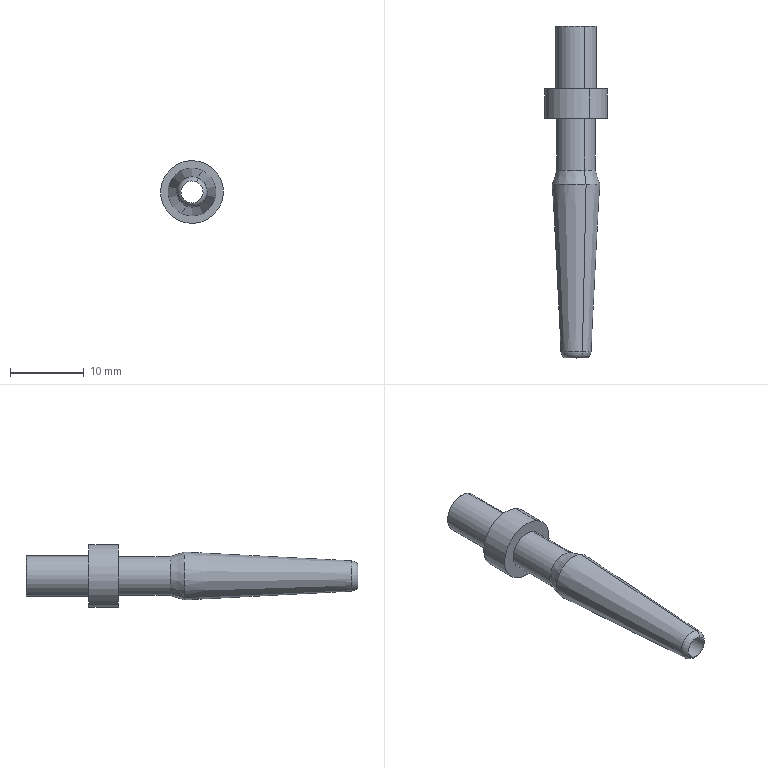Component | SolidWorks | WireFeedingNozzle-1 | 1 solid | 19 faces | box 8.5 x 44.89 x 8.5 mm | volume 831 mm3 | cylinder 8 | cone 6 | plane 3 | torus 2 | commonest cylinder face diameters 3 x2 5.5 x2 8.5 x2 5.274 x2
build123d program:
from build123d import *

# Parameters (mm, degrees)
FILLET3_R          = 1
CUT_EXTRUDE1_REACH = 47.4
SKETCH2_R          = 1.5
CHAMFER1_SIZE      = 0.08


with BuildPart() as part:
    # Sketch1 → Revolve1 (revolve)
    with BuildSketch(Plane.XY, mode=Mode.PRIVATE) as revolve1_sk:
        Polygon((-15.381, 0), (29.619, 0), (29.619, 2), (6.04, 3.236), (4.119, 2.637), (-2.881, 2.637), (-2.881, 4.25), (-6.881, 4.25), (-6.881, 2.75), (-15.381, 2.75), align=None)
    revolve(revolve1_sk.sketch.rotate(Axis((-15.381, 0, 0), (1, 0, 0)), 90), axis=Axis((-15.381, 0, 0), (1, 0, 0)))

    # Fillet3
    fillet3_edges = [part.edges().sort_by_distance(p)[0] for p in [
        (29.619, 0, -2),
    ]]
    fillet(fillet3_edges, radius=FILLET3_R)

    # Sketch2 → Cut-Extrude1 (cut, up to next)
    with BuildSketch(Plane.ZY.offset(15.381), mode=Mode.PRIVATE) as cut_extrude1_sk1:
        Circle(SKETCH2_R)
    cut_extrude1_tool1 = extrude(cut_extrude1_sk1.sketch, amount=-CUT_EXTRUDE1_REACH, mode=Mode.PRIVATE) & part.part
    add(cut_extrude1_tool1.solids().sort_by_distance((-15.381, 0, 0))[0], mode=Mode.SUBTRACT)

    # Chamfer1
    chamfer1_edges = [part.edges().sort_by_distance(p)[0] for p in [
        (-15.381, 0, -2.75),
    ]]
    chamfer(chamfer1_edges, length=CHAMFER1_SIZE)


solid = part.part

# Placed as in the assembly
solid = solid.moved(Location((-5.981, -114.875, 160), (0, 0, -90)))
STEP:
#1=CARTESIAN_POINT('',(-0.1912,-3.917,6.395));
#2=VERTEX_POINT('',#1);
#3=CARTESIAN_POINT('',(-0.2797,-3.917,6.204));
#4=VERTEX_POINT('',#3);
#5=CARTESIAN_POINT('',(-0.2355,-3.917,6.299));
#6=DIRECTION('',(0.,1.,0.));
#7=DIRECTION('',(-0.421,0.,-0.9071));
#8=AXIS2_PLACEMENT_3D('',#5,#6,#7);
#9=CIRCLE('',#8,0.1051);
#10=EDGE_CURVE('',#2,#4,#9,.T.);
#11=ORIENTED_EDGE('',*,*,#10,.F.);
#12=CARTESIAN_POINT('',(-0.1899,-3.92,6.397));
#13=VERTEX_POINT('',#12);
#14=CARTESIAN_POINT('',(-0.1912,-3.917,6.395));
#15=DIRECTION('',(0.2977,-0.7071,0.6414));
#16=VECTOR('',#15,39.37);
#17=LINE('',#14,#16);
#18=EDGE_CURVE('',#2,#13,#17,.T.);
#19=ORIENTED_EDGE('',*,*,#18,.T.);
#20=CARTESIAN_POINT('',(-0.281,-3.92,6.201));
#21=VERTEX_POINT('',#20);
#22=CARTESIAN_POINT('',(-0.2355,-3.92,6.299));
#23=DIRECTION('',(-0.,-1.,-0.));
#24=DIRECTION('',(-0.421,0.,-0.9071));
#25=AXIS2_PLACEMENT_3D('',#22,#23,#24);
#26=CIRCLE('',#25,0.1083);
#27=EDGE_CURVE('',#21,#13,#26,.T.);
#28=ORIENTED_EDGE('',*,*,#27,.F.);
#29=CARTESIAN_POINT('',(-0.2797,-3.917,6.204));
#30=DIRECTION('',(-0.2977,-0.7071,-0.6414));
#31=VECTOR('',#30,39.37);
#32=LINE('',#29,#31);
#33=EDGE_CURVE('',#4,#21,#32,.T.);
#34=ORIENTED_EDGE('',*,*,#33,.F.);
#35=EDGE_LOOP('',(#11,#19,#28,#34));
#36=FACE_OUTER_BOUND('',#35,.T.);
#37=CARTESIAN_POINT('',(-0.2355,-3.917,6.299));
#38=DIRECTION('',(-0.,-1.,-0.));
#39=DIRECTION('',(-0.421,0.,-0.9071));
#40=AXIS2_PLACEMENT_3D('',#37,#38,#39);
#41=CONICAL_SURFACE('',#40,0.1051,0.7854);
#42=ADVANCED_FACE('',(#36),#41,.T.);
#43=CARTESIAN_POINT('',(-0.2603,-5.685,6.246));
#44=VERTEX_POINT('',#43);
#45=CARTESIAN_POINT('',(-0.2106,-5.685,6.353));
#46=VERTEX_POINT('',#45);
#47=CARTESIAN_POINT('',(-0.2355,-5.685,6.299));
#48=DIRECTION('',(0.,1.,0.));
#49=DIRECTION('',(0.421,0.,0.9071));
#50=AXIS2_PLACEMENT_3D('',#47,#48,#49);
#51=CIRCLE('',#50,0.05906);
#52=EDGE_CURVE('',#44,#46,#51,.T.);
#53=ORIENTED_EDGE('',*,*,#52,.F.);
#54=CARTESIAN_POINT('',(-0.2603,-3.917,6.246));
#55=VERTEX_POINT('',#54);
#56=CARTESIAN_POINT('',(-0.2603,-5.689,6.246));
#57=DIRECTION('',(0.,1.,0.));
#58=VECTOR('',#57,39.37);
#59=LINE('',#56,#58);
#60=EDGE_CURVE('',#44,#55,#59,.T.);
#61=ORIENTED_EDGE('',*,*,#60,.T.);
#62=CARTESIAN_POINT('',(-0.2106,-3.917,6.353));
#63=VERTEX_POINT('',#62);
#64=CARTESIAN_POINT('',(-0.2355,-3.917,6.299));
#65=DIRECTION('',(0.,1.,0.));
#66=DIRECTION('',(0.421,0.,0.9071));
#67=AXIS2_PLACEMENT_3D('',#64,#65,#66);
#68=CIRCLE('',#67,0.05906);
#69=EDGE_CURVE('',#55,#63,#68,.T.);
#70=ORIENTED_EDGE('',*,*,#69,.T.);
#71=CARTESIAN_POINT('',(-0.2106,-5.689,6.353));
#72=DIRECTION('',(0.,1.,0.));
#73=VECTOR('',#72,39.37);
#74=LINE('',#71,#73);
#75=EDGE_CURVE('',#46,#63,#74,.T.);
#76=ORIENTED_EDGE('',*,*,#75,.F.);
#77=EDGE_LOOP('',(#53,#61,#70,#76));
#78=FACE_OUTER_BOUND('',#77,.T.);
#79=CARTESIAN_POINT('',(-0.2355,-5.689,6.299));
#80=DIRECTION('',(0.,1.,0.));
#81=DIRECTION('',(0.421,0.,0.9071));
#82=AXIS2_PLACEMENT_3D('',#79,#80,#81);
#83=CYLINDRICAL_SURFACE('',#82,0.05906);
#84=ADVANCED_FACE('',(#78),#83,.F.);
#85=CARTESIAN_POINT('',(-0.2355,-5.685,6.299));
#86=DIRECTION('',(0.,1.,0.));
#87=DIRECTION('',(0.421,0.,0.9071));
#88=AXIS2_PLACEMENT_3D('',#85,#86,#87);
#89=CIRCLE('',#88,0.05906);
#90=EDGE_CURVE('',#46,#44,#89,.T.);
#91=ORIENTED_EDGE('',*,*,#90,.T.);
#92=CARTESIAN_POINT('',(-0.2694,-5.651,6.226));
#93=VERTEX_POINT('',#92);
#94=CARTESIAN_POINT('',(-0.2529,-5.649,6.262));
#95=DIRECTION('',(0.9071,-0.,-0.421));
#96=DIRECTION('',(-0.421,0.,-0.9071));
#97=AXIS2_PLACEMENT_3D('',#94,#95,#96);
#98=CIRCLE('',#97,0.03937);
#99=EDGE_CURVE('',#44,#93,#98,.T.);
#100=ORIENTED_EDGE('',*,*,#99,.T.);
#101=CARTESIAN_POINT('',(-0.2015,-5.651,6.372));
#102=VERTEX_POINT('',#101);
#103=CARTESIAN_POINT('',(-0.2355,-5.651,6.299));
#104=DIRECTION('',(0.,1.,0.));
#105=DIRECTION('',(-0.421,0.,-0.9071));
#106=AXIS2_PLACEMENT_3D('',#103,#104,#105);
#107=CIRCLE('',#106,0.0807);
#108=EDGE_CURVE('',#102,#93,#107,.T.);
#109=ORIENTED_EDGE('',*,*,#108,.F.);
#110=CARTESIAN_POINT('',(-0.218,-5.649,6.337));
#111=DIRECTION('',(-0.9071,0.,0.421));
#112=DIRECTION('',(0.421,0.,0.9071));
#113=AXIS2_PLACEMENT_3D('',#110,#111,#112);
#114=CIRCLE('',#113,0.03937);
#115=EDGE_CURVE('',#46,#102,#114,.T.);
#116=ORIENTED_EDGE('',*,*,#115,.F.);
#117=EDGE_LOOP('',(#91,#100,#109,#116));
#118=FACE_OUTER_BOUND('',#117,.T.);
#119=CARTESIAN_POINT('',(-0.2355,-5.649,6.299));
#120=DIRECTION('',(0.,1.,0.));
#121=DIRECTION('',(0.421,-0.,0.9071));
#122=AXIS2_PLACEMENT_3D('',#119,#120,#121);
#123=TOROIDAL_SURFACE('',#122,0.04138,0.03937);
#124=ADVANCED_FACE('',(#118),#123,.T.);
#125=CARTESIAN_POINT('',(-0.1899,-4.252,6.397));
#126=VERTEX_POINT('',#125);
#127=CARTESIAN_POINT('',(-0.281,-4.252,6.201));
#128=VERTEX_POINT('',#127);
#129=CARTESIAN_POINT('',(-0.2355,-4.252,6.299));
#130=DIRECTION('',(0.,1.,0.));
#131=DIRECTION('',(0.421,0.,0.9071));
#132=AXIS2_PLACEMENT_3D('',#129,#130,#131);
#133=CIRCLE('',#132,0.1083);
#134=EDGE_CURVE('',#126,#128,#133,.T.);
#135=ORIENTED_EDGE('',*,*,#134,.T.);
#136=CARTESIAN_POINT('',(-0.281,-3.917,6.201));
#137=DIRECTION('',(0.,1.,0.));
#138=VECTOR('',#137,39.37);
#139=LINE('',#136,#138);
#140=EDGE_CURVE('',#128,#21,#139,.T.);
#141=ORIENTED_EDGE('',*,*,#140,.T.);
#142=ORIENTED_EDGE('',*,*,#27,.T.);
#143=CARTESIAN_POINT('',(-0.1899,-3.917,6.397));
#144=DIRECTION('',(0.,1.,0.));
#145=VECTOR('',#144,39.37);
#146=LINE('',#143,#145);
#147=EDGE_CURVE('',#126,#13,#146,.T.);
#148=ORIENTED_EDGE('',*,*,#147,.F.);
#149=EDGE_LOOP('',(#135,#141,#142,#148));
#150=FACE_OUTER_BOUND('',#149,.T.);
#151=CARTESIAN_POINT('',(-0.2355,-3.917,6.299));
#152=DIRECTION('',(0.,1.,0.));
#153=DIRECTION('',(0.421,0.,0.9071));
#154=AXIS2_PLACEMENT_3D('',#151,#152,#153);
#155=CYLINDRICAL_SURFACE('',#154,0.1083);
#156=ADVANCED_FACE('',(#150),#155,.T.);
#157=CARTESIAN_POINT('',(-0.165,-4.409,6.451));
#158=VERTEX_POINT('',#157);
#159=CARTESIAN_POINT('',(-0.3059,-4.409,6.147));
#160=VERTEX_POINT('',#159);
#161=CARTESIAN_POINT('',(-0.2355,-4.409,6.299));
#162=DIRECTION('',(0.,1.,0.));
#163=DIRECTION('',(0.421,0.,0.9071));
#164=AXIS2_PLACEMENT_3D('',#161,#162,#163);
#165=CIRCLE('',#164,0.1673);
#166=EDGE_CURVE('',#158,#160,#165,.T.);
#167=ORIENTED_EDGE('',*,*,#166,.T.);
#168=CARTESIAN_POINT('',(-0.3059,-4.252,6.147));
#169=VERTEX_POINT('',#168);
#170=CARTESIAN_POINT('',(-0.3059,-3.917,6.147));
#171=DIRECTION('',(0.,1.,0.));
#172=VECTOR('',#171,39.37);
#173=LINE('',#170,#172);
#174=EDGE_CURVE('',#160,#169,#173,.T.);
#175=ORIENTED_EDGE('',*,*,#174,.T.);
#176=CARTESIAN_POINT('',(-0.165,-4.252,6.451));
#177=VERTEX_POINT('',#176);
#178=CARTESIAN_POINT('',(-0.2355,-4.252,6.299));
#179=DIRECTION('',(0.,1.,0.));
#180=DIRECTION('',(0.421,0.,0.9071));
#181=AXIS2_PLACEMENT_3D('',#178,#179,#180);
#182=CIRCLE('',#181,0.1673);
#183=EDGE_CURVE('',#177,#169,#182,.T.);
#184=ORIENTED_EDGE('',*,*,#183,.F.);
#185=CARTESIAN_POINT('',(-0.165,-3.917,6.451));
#186=DIRECTION('',(0.,1.,0.));
#187=VECTOR('',#186,39.37);
#188=LINE('',#185,#187);
#189=EDGE_CURVE('',#158,#177,#188,.T.);
#190=ORIENTED_EDGE('',*,*,#189,.F.);
#191=EDGE_LOOP('',(#167,#175,#184,#190));
#192=FACE_OUTER_BOUND('',#191,.T.);
#193=CARTESIAN_POINT('',(-0.2355,-3.917,6.299));
#194=DIRECTION('',(0.,1.,0.));
#195=DIRECTION('',(0.421,0.,0.9071));
#196=AXIS2_PLACEMENT_3D('',#193,#194,#195);
#197=CYLINDRICAL_SURFACE('',#196,0.1673);
#198=ADVANCED_FACE('',(#192),#197,.T.);
#199=CARTESIAN_POINT('',(-0.1918,-4.685,6.393));
#200=VERTEX_POINT('',#199);
#201=CARTESIAN_POINT('',(-0.2792,-4.685,6.205));
#202=VERTEX_POINT('',#201);
#203=CARTESIAN_POINT('',(-0.2355,-4.685,6.299));
#204=DIRECTION('',(0.,1.,0.));
#205=DIRECTION('',(0.421,0.,0.9071));
#206=AXIS2_PLACEMENT_3D('',#203,#204,#205);
#207=CIRCLE('',#206,0.1038);
#208=EDGE_CURVE('',#200,#202,#207,.T.);
#209=ORIENTED_EDGE('',*,*,#208,.T.);
#210=CARTESIAN_POINT('',(-0.2792,-4.409,6.205));
#211=VERTEX_POINT('',#210);
#212=CARTESIAN_POINT('',(-0.2792,-3.917,6.205));
#213=DIRECTION('',(0.,1.,0.));
#214=VECTOR('',#213,39.37);
#215=LINE('',#212,#214);
#216=EDGE_CURVE('',#202,#211,#215,.T.);
#217=ORIENTED_EDGE('',*,*,#216,.T.);
#218=CARTESIAN_POINT('',(-0.1918,-4.409,6.393));
#219=VERTEX_POINT('',#218);
#220=CARTESIAN_POINT('',(-0.2355,-4.409,6.299));
#221=DIRECTION('',(0.,1.,0.));
#222=DIRECTION('',(0.421,0.,0.9071));
#223=AXIS2_PLACEMENT_3D('',#220,#221,#222);
#224=CIRCLE('',#223,0.1038);
#225=EDGE_CURVE('',#219,#211,#224,.T.);
#226=ORIENTED_EDGE('',*,*,#225,.F.);
#227=CARTESIAN_POINT('',(-0.1918,-3.917,6.393));
#228=DIRECTION('',(0.,1.,0.));
#229=VECTOR('',#228,39.37);
#230=LINE('',#227,#229);
#231=EDGE_CURVE('',#200,#219,#230,.T.);
#232=ORIENTED_EDGE('',*,*,#231,.F.);
#233=EDGE_LOOP('',(#209,#217,#226,#232));
#234=FACE_OUTER_BOUND('',#233,.T.);
#235=CARTESIAN_POINT('',(-0.2355,-3.917,6.299));
#236=DIRECTION('',(0.,1.,0.));
#237=DIRECTION('',(0.421,0.,0.9071));
#238=AXIS2_PLACEMENT_3D('',#235,#236,#237);
#239=CYLINDRICAL_SURFACE('',#238,0.1038);
#240=ADVANCED_FACE('',(#234),#239,.T.);
#241=ORIENTED_EDGE('',*,*,#208,.F.);
#242=CARTESIAN_POINT('',(-0.1818,-4.76,6.415));
#243=VERTEX_POINT('',#242);
#244=CARTESIAN_POINT('',(-0.1818,-4.76,6.415));
#245=DIRECTION('',(0.1253,-0.9547,0.27));
#246=VECTOR('',#245,39.37);
#247=LINE('',#244,#246);
#248=EDGE_CURVE('',#200,#243,#247,.T.);
#249=ORIENTED_EDGE('',*,*,#248,.T.);
#250=CARTESIAN_POINT('',(-0.2891,-4.76,6.184));
#251=VERTEX_POINT('',#250);
#252=CARTESIAN_POINT('',(-0.2355,-4.76,6.299));
#253=DIRECTION('',(0.,1.,0.));
#254=DIRECTION('',(0.421,0.,0.9071));
#255=AXIS2_PLACEMENT_3D('',#252,#253,#254);
#256=CIRCLE('',#255,0.1274);
#257=EDGE_CURVE('',#243,#251,#256,.T.);
#258=ORIENTED_EDGE('',*,*,#257,.T.);
#259=CARTESIAN_POINT('',(-0.2891,-4.76,6.184));
#260=DIRECTION('',(-0.1253,-0.9547,-0.27));
#261=VECTOR('',#260,39.37);
#262=LINE('',#259,#261);
#263=EDGE_CURVE('',#202,#251,#262,.T.);
#264=ORIENTED_EDGE('',*,*,#263,.F.);
#265=EDGE_LOOP('',(#241,#249,#258,#264));
#266=FACE_OUTER_BOUND('',#265,.T.);
#267=CARTESIAN_POINT('',(-0.2355,-4.76,6.299));
#268=DIRECTION('',(-0.,-1.,-0.));
#269=DIRECTION('',(-0.421,0.,-0.9071));
#270=AXIS2_PLACEMENT_3D('',#267,#268,#269);
#271=CONICAL_SURFACE('',#270,0.1274,0.3023);
#272=ADVANCED_FACE('',(#266),#271,.T.);
#273=ORIENTED_EDGE('',*,*,#108,.T.);
#274=CARTESIAN_POINT('',(-0.2686,-5.689,6.228));
#275=DIRECTION('',(-0.02203,0.9986,-0.04747));
#276=VECTOR('',#275,39.37);
#277=LINE('',#274,#276);
#278=EDGE_CURVE('',#93,#251,#277,.T.);
#279=ORIENTED_EDGE('',*,*,#278,.T.);
#280=ORIENTED_EDGE('',*,*,#257,.F.);
#281=CARTESIAN_POINT('',(-0.2023,-5.689,6.371));
#282=DIRECTION('',(0.02203,0.9986,0.04747));
#283=VECTOR('',#282,39.37);
#284=LINE('',#281,#283);
#285=EDGE_CURVE('',#102,#243,#284,.T.);
#286=ORIENTED_EDGE('',*,*,#285,.F.);
#287=EDGE_LOOP('',(#273,#279,#280,#286));
#288=FACE_OUTER_BOUND('',#287,.T.);
#289=CARTESIAN_POINT('',(-0.2355,-5.689,6.299));
#290=DIRECTION('',(0.,1.,0.));
#291=DIRECTION('',(0.421,0.,0.9071));
#292=AXIS2_PLACEMENT_3D('',#289,#290,#291);
#293=CONICAL_SURFACE('',#292,0.07874,0.05236);
#294=ADVANCED_FACE('',(#288),#293,.T.);
#295=CARTESIAN_POINT('',(-0.2355,-3.917,6.299));
#296=DIRECTION('',(0.,1.,0.));
#297=DIRECTION('',(-0.421,0.,-0.9071));
#298=AXIS2_PLACEMENT_3D('',#295,#296,#297);
#299=CIRCLE('',#298,0.1051);
#300=EDGE_CURVE('',#4,#2,#299,.T.);
#301=ORIENTED_EDGE('',*,*,#300,.T.);
#302=ORIENTED_EDGE('',*,*,#10,.T.);
#303=EDGE_LOOP('',(#301,#302));
#304=FACE_OUTER_BOUND('',#303,.T.);
#305=CARTESIAN_POINT('',(-0.2355,-3.917,6.299));
#306=DIRECTION('',(0.,1.,0.));
#307=DIRECTION('',(0.421,0.,0.9071));
#308=AXIS2_PLACEMENT_3D('',#305,#306,#307);
#309=CIRCLE('',#308,0.05906);
#310=EDGE_CURVE('',#63,#55,#309,.T.);
#311=ORIENTED_EDGE('',*,*,#310,.F.);
#312=ORIENTED_EDGE('',*,*,#69,.F.);
#313=EDGE_LOOP('',(#311,#312));
#314=FACE_BOUND('',#313,.T.);
#315=CARTESIAN_POINT('',(-0.1373,-3.917,6.254));
#316=DIRECTION('',(-0.,-1.,-0.));
#317=DIRECTION('',(-0.421,0.,-0.9071));
#318=AXIS2_PLACEMENT_3D('',#315,#316,#317);
#319=PLANE('',#318);
#320=ADVANCED_FACE('',(#304,#314),#319,.F.);
#321=ORIENTED_EDGE('',*,*,#278,.F.);
#322=CARTESIAN_POINT('',(-0.2355,-5.651,6.299));
#323=DIRECTION('',(0.,1.,0.));
#324=DIRECTION('',(-0.421,0.,-0.9071));
#325=AXIS2_PLACEMENT_3D('',#322,#323,#324);
#326=CIRCLE('',#325,0.0807);
#327=EDGE_CURVE('',#93,#102,#326,.T.);
#328=ORIENTED_EDGE('',*,*,#327,.T.);
#329=ORIENTED_EDGE('',*,*,#285,.T.);
#330=CARTESIAN_POINT('',(-0.2355,-4.76,6.299));
#331=DIRECTION('',(0.,1.,0.));
#332=DIRECTION('',(0.421,0.,0.9071));
#333=AXIS2_PLACEMENT_3D('',#330,#331,#332);
#334=CIRCLE('',#333,0.1274);
#335=EDGE_CURVE('',#251,#243,#334,.T.);
#336=ORIENTED_EDGE('',*,*,#335,.F.);
#337=EDGE_LOOP('',(#321,#328,#329,#336));
#338=FACE_OUTER_BOUND('',#337,.T.);
#339=CARTESIAN_POINT('',(-0.2355,-5.689,6.299));
#340=DIRECTION('',(0.,1.,0.));
#341=DIRECTION('',(0.421,0.,0.9071));
#342=AXIS2_PLACEMENT_3D('',#339,#340,#341);
#343=CONICAL_SURFACE('',#342,0.07874,0.05236);
#344=ADVANCED_FACE('',(#338),#343,.T.);
#345=ORIENTED_EDGE('',*,*,#248,.F.);
#346=CARTESIAN_POINT('',(-0.2355,-4.685,6.299));
#347=DIRECTION('',(0.,1.,0.));
#348=DIRECTION('',(0.421,0.,0.9071));
#349=AXIS2_PLACEMENT_3D('',#346,#347,#348);
#350=CIRCLE('',#349,0.1038);
#351=EDGE_CURVE('',#202,#200,#350,.T.);
#352=ORIENTED_EDGE('',*,*,#351,.F.);
#353=ORIENTED_EDGE('',*,*,#263,.T.);
#354=ORIENTED_EDGE('',*,*,#335,.T.);
#355=EDGE_LOOP('',(#345,#352,#353,#354));
#356=FACE_OUTER_BOUND('',#355,.T.);
#357=CARTESIAN_POINT('',(-0.2355,-4.76,6.299));
#358=DIRECTION('',(-0.,-1.,-0.));
#359=DIRECTION('',(-0.421,0.,-0.9071));
#360=AXIS2_PLACEMENT_3D('',#357,#358,#359);
#361=CONICAL_SURFACE('',#360,0.1274,0.3023);
#362=ADVANCED_FACE('',(#356),#361,.T.);
#363=ORIENTED_EDGE('',*,*,#216,.F.);
#364=ORIENTED_EDGE('',*,*,#351,.T.);
#365=ORIENTED_EDGE('',*,*,#231,.T.);
#366=CARTESIAN_POINT('',(-0.2355,-4.409,6.299));
#367=DIRECTION('',(0.,1.,0.));
#368=DIRECTION('',(0.421,0.,0.9071));
#369=AXIS2_PLACEMENT_3D('',#366,#367,#368);
#370=CIRCLE('',#369,0.1038);
#371=EDGE_CURVE('',#211,#219,#370,.T.);
#372=ORIENTED_EDGE('',*,*,#371,.F.);
#373=EDGE_LOOP('',(#363,#364,#365,#372));
#374=FACE_OUTER_BOUND('',#373,.T.);
#375=CARTESIAN_POINT('',(-0.2355,-3.917,6.299));
#376=DIRECTION('',(0.,1.,0.));
#377=DIRECTION('',(0.421,0.,0.9071));
#378=AXIS2_PLACEMENT_3D('',#375,#376,#377);
#379=CYLINDRICAL_SURFACE('',#378,0.1038);
#380=ADVANCED_FACE('',(#374),#379,.T.);
#381=ORIENTED_EDGE('',*,*,#166,.F.);
#382=CARTESIAN_POINT('',(-0.2355,-4.409,6.299));
#383=DIRECTION('',(0.,1.,0.));
#384=DIRECTION('',(0.421,0.,0.9071));
#385=AXIS2_PLACEMENT_3D('',#382,#383,#384);
#386=CIRCLE('',#385,0.1673);
#387=EDGE_CURVE('',#160,#158,#386,.T.);
#388=ORIENTED_EDGE('',*,*,#387,.F.);
#389=EDGE_LOOP('',(#381,#388));
#390=FACE_OUTER_BOUND('',#389,.T.);
#391=ORIENTED_EDGE('',*,*,#225,.T.);
#392=ORIENTED_EDGE('',*,*,#371,.T.);
#393=EDGE_LOOP('',(#391,#392));
#394=FACE_BOUND('',#393,.T.);
#395=CARTESIAN_POINT('',(-0.1413,-4.409,6.256));
#396=DIRECTION('',(0.,1.,0.));
#397=DIRECTION('',(0.421,-0.,0.9071));
#398=AXIS2_PLACEMENT_3D('',#395,#396,#397);
#399=PLANE('',#398);
#400=ADVANCED_FACE('',(#390,#394),#399,.F.);
#401=ORIENTED_EDGE('',*,*,#174,.F.);
#402=ORIENTED_EDGE('',*,*,#387,.T.);
#403=ORIENTED_EDGE('',*,*,#189,.T.);
#404=CARTESIAN_POINT('',(-0.2355,-4.252,6.299));
#405=DIRECTION('',(0.,1.,0.));
#406=DIRECTION('',(0.421,0.,0.9071));
#407=AXIS2_PLACEMENT_3D('',#404,#405,#406);
#408=CIRCLE('',#407,0.1673);
#409=EDGE_CURVE('',#169,#177,#408,.T.);
#410=ORIENTED_EDGE('',*,*,#409,.F.);
#411=EDGE_LOOP('',(#401,#402,#403,#410));
#412=FACE_OUTER_BOUND('',#411,.T.);
#413=CARTESIAN_POINT('',(-0.2355,-3.917,6.299));
#414=DIRECTION('',(0.,1.,0.));
#415=DIRECTION('',(0.421,0.,0.9071));
#416=AXIS2_PLACEMENT_3D('',#413,#414,#415);
#417=CYLINDRICAL_SURFACE('',#416,0.1673);
#418=ADVANCED_FACE('',(#412),#417,.T.);
#419=ORIENTED_EDGE('',*,*,#134,.F.);
#420=CARTESIAN_POINT('',(-0.2355,-4.252,6.299));
#421=DIRECTION('',(0.,1.,0.));
#422=DIRECTION('',(0.421,0.,0.9071));
#423=AXIS2_PLACEMENT_3D('',#420,#421,#422);
#424=CIRCLE('',#423,0.1083);
#425=EDGE_CURVE('',#128,#126,#424,.T.);
#426=ORIENTED_EDGE('',*,*,#425,.F.);
#427=EDGE_LOOP('',(#419,#426));
#428=FACE_BOUND('',#427,.T.);
#429=ORIENTED_EDGE('',*,*,#183,.T.);
#430=ORIENTED_EDGE('',*,*,#409,.T.);
#431=EDGE_LOOP('',(#429,#430));
#432=FACE_OUTER_BOUND('',#431,.T.);
#433=CARTESIAN_POINT('',(-0.0837,-4.252,6.229));
#434=DIRECTION('',(-0.,-1.,-0.));
#435=DIRECTION('',(-0.421,0.,-0.9071));
#436=AXIS2_PLACEMENT_3D('',#433,#434,#435);
#437=PLANE('',#436);
#438=ADVANCED_FACE('',(#428,#432),#437,.F.);
#439=ORIENTED_EDGE('',*,*,#140,.F.);
#440=ORIENTED_EDGE('',*,*,#425,.T.);
#441=ORIENTED_EDGE('',*,*,#147,.T.);
#442=CARTESIAN_POINT('',(-0.2355,-3.92,6.299));
#443=DIRECTION('',(-0.,-1.,-0.));
#444=DIRECTION('',(-0.421,0.,-0.9071));
#445=AXIS2_PLACEMENT_3D('',#442,#443,#444);
#446=CIRCLE('',#445,0.1083);
#447=EDGE_CURVE('',#13,#21,#446,.T.);
#448=ORIENTED_EDGE('',*,*,#447,.T.);
#449=EDGE_LOOP('',(#439,#440,#441,#448));
#450=FACE_OUTER_BOUND('',#449,.T.);
#451=CARTESIAN_POINT('',(-0.2355,-3.917,6.299));
#452=DIRECTION('',(0.,1.,0.));
#453=DIRECTION('',(0.421,0.,0.9071));
#454=AXIS2_PLACEMENT_3D('',#451,#452,#453);
#455=CYLINDRICAL_SURFACE('',#454,0.1083);
#456=ADVANCED_FACE('',(#450),#455,.T.);
#457=ORIENTED_EDGE('',*,*,#99,.F.);
#458=ORIENTED_EDGE('',*,*,#52,.T.);
#459=ORIENTED_EDGE('',*,*,#115,.T.);
#460=ORIENTED_EDGE('',*,*,#327,.F.);
#461=EDGE_LOOP('',(#457,#458,#459,#460));
#462=FACE_OUTER_BOUND('',#461,.T.);
#463=CARTESIAN_POINT('',(-0.2355,-5.649,6.299));
#464=DIRECTION('',(0.,1.,0.));
#465=DIRECTION('',(0.421,-0.,0.9071));
#466=AXIS2_PLACEMENT_3D('',#463,#464,#465);
#467=TOROIDAL_SURFACE('',#466,0.04138,0.03937);
#468=ADVANCED_FACE('',(#462),#467,.T.);
#469=ORIENTED_EDGE('',*,*,#60,.F.);
#470=ORIENTED_EDGE('',*,*,#90,.F.);
#471=ORIENTED_EDGE('',*,*,#75,.T.);
#472=ORIENTED_EDGE('',*,*,#310,.T.);
#473=EDGE_LOOP('',(#469,#470,#471,#472));
#474=FACE_OUTER_BOUND('',#473,.T.);
#475=CARTESIAN_POINT('',(-0.2355,-5.689,6.299));
#476=DIRECTION('',(0.,1.,0.));
#477=DIRECTION('',(0.421,0.,0.9071));
#478=AXIS2_PLACEMENT_3D('',#475,#476,#477);
#479=CYLINDRICAL_SURFACE('',#478,0.05906);
#480=ADVANCED_FACE('',(#474),#479,.F.);
#481=ORIENTED_EDGE('',*,*,#18,.F.);
#482=ORIENTED_EDGE('',*,*,#300,.F.);
#483=ORIENTED_EDGE('',*,*,#33,.T.);
#484=ORIENTED_EDGE('',*,*,#447,.F.);
#485=EDGE_LOOP('',(#481,#482,#483,#484));
#486=FACE_OUTER_BOUND('',#485,.T.);
#487=CARTESIAN_POINT('',(-0.2355,-3.917,6.299));
#488=DIRECTION('',(-0.,-1.,-0.));
#489=DIRECTION('',(-0.421,0.,-0.9071));
#490=AXIS2_PLACEMENT_3D('',#487,#488,#489);
#491=CONICAL_SURFACE('',#490,0.1051,0.7854);
#492=ADVANCED_FACE('',(#486),#491,.T.);
#493=CLOSED_SHELL('',(#42,#84,#124,#156,#198,#240,#272,#294,#320,#344,#362,#380,#400,#418,#438,#456,#468,#480,#492));
#494=MANIFOLD_SOLID_BREP('',#493);
#495=CARTESIAN_POINT('',(0.,0.,0.));
#496=DIRECTION('',(0.,0.,1.));
#497=DIRECTION('',(1.,0.,0.));
#498=AXIS2_PLACEMENT_3D('',#495,#496,#497);
#499=(LENGTH_UNIT()NAMED_UNIT(*)SI_UNIT($,.METRE.));
#500=LENGTH_MEASURE_WITH_UNIT(LENGTH_MEASURE(0.0254),#499);
#501=DIMENSIONAL_EXPONENTS(1.,0.,0.,0.,0.,0.,0.);
#502=(CONVERSION_BASED_UNIT('',#500)LENGTH_UNIT()NAMED_UNIT(#501));
#503=UNCERTAINTY_MEASURE_WITH_UNIT(LENGTH_MEASURE(0.00001),#502,'','');
#504=(NAMED_UNIT(*)PLANE_ANGLE_UNIT()SI_UNIT($,.RADIAN.));
#505=(NAMED_UNIT(*)SI_UNIT($,.STERADIAN.)SOLID_ANGLE_UNIT());
#506=(GEOMETRIC_REPRESENTATION_CONTEXT(3)GLOBAL_UNCERTAINTY_ASSIGNED_CONTEXT((#503))GLOBAL_UNIT_ASSIGNED_CONTEXT((#502,#504,#505))REPRESENTATION_CONTEXT('',''));
#507=ADVANCED_BREP_SHAPE_REPRESENTATION('',(#494,#498),#506);
#508=COLOUR_RGB('',0.7922,0.8196,0.9333);
#509=FILL_AREA_STYLE_COLOUR('',#508);
#510=FILL_AREA_STYLE('',(#509));
#511=SURFACE_STYLE_FILL_AREA(#510);
#512=SURFACE_SIDE_STYLE('',(#511));
#513=SURFACE_STYLE_USAGE(.BOTH.,#512);
#514=PRESENTATION_STYLE_ASSIGNMENT((#513));
#515=STYLED_ITEM('',(#514),#494);
#516=PRESENTATION_LAYER_ASSIGNMENT('','',(#515));
#517=(LENGTH_UNIT()NAMED_UNIT(*)SI_UNIT($,.METRE.));
#518=LENGTH_MEASURE_WITH_UNIT(LENGTH_MEASURE(0.0254),#517);
#519=DIMENSIONAL_EXPONENTS(1.,0.,0.,0.,0.,0.,0.);
#520=(CONVERSION_BASED_UNIT('',#518)LENGTH_UNIT()NAMED_UNIT(#519));
#521=UNCERTAINTY_MEASURE_WITH_UNIT(LENGTH_MEASURE(0.00001),#520,'','');
#522=(NAMED_UNIT(*)PLANE_ANGLE_UNIT()SI_UNIT($,.RADIAN.));
#523=(NAMED_UNIT(*)SI_UNIT($,.STERADIAN.)SOLID_ANGLE_UNIT());
#524=(GEOMETRIC_REPRESENTATION_CONTEXT(3)GLOBAL_UNCERTAINTY_ASSIGNED_CONTEXT((#521))GLOBAL_UNIT_ASSIGNED_CONTEXT((#520,#522,#523))REPRESENTATION_CONTEXT('',''));
#525=MECHANICAL_DESIGN_GEOMETRIC_PRESENTATION_REPRESENTATION('',(#515),#524);